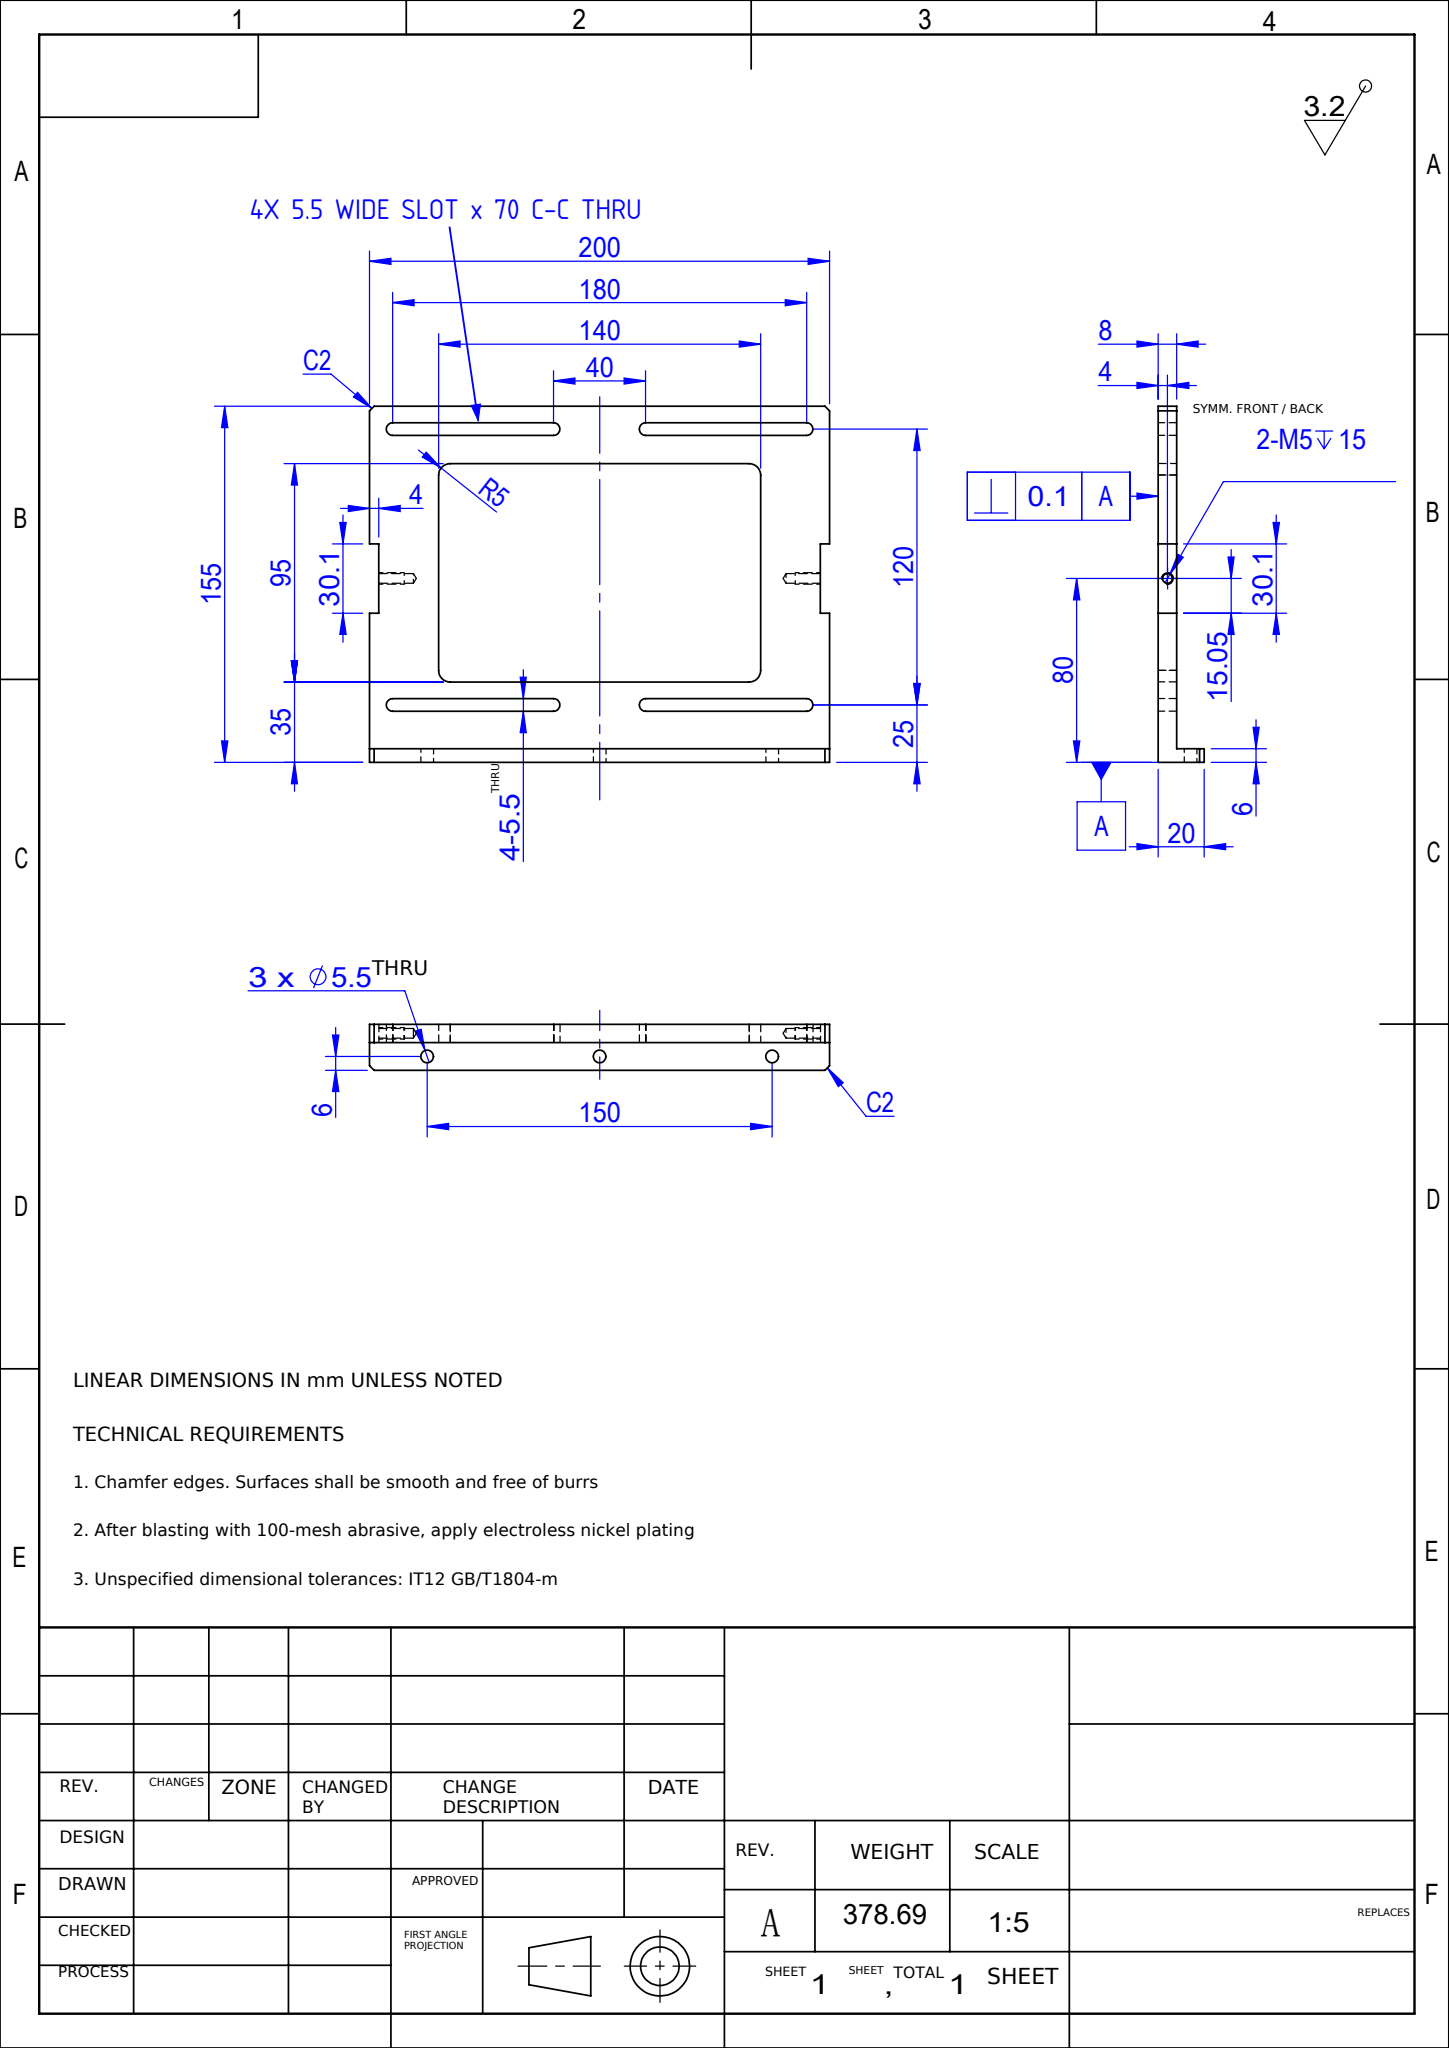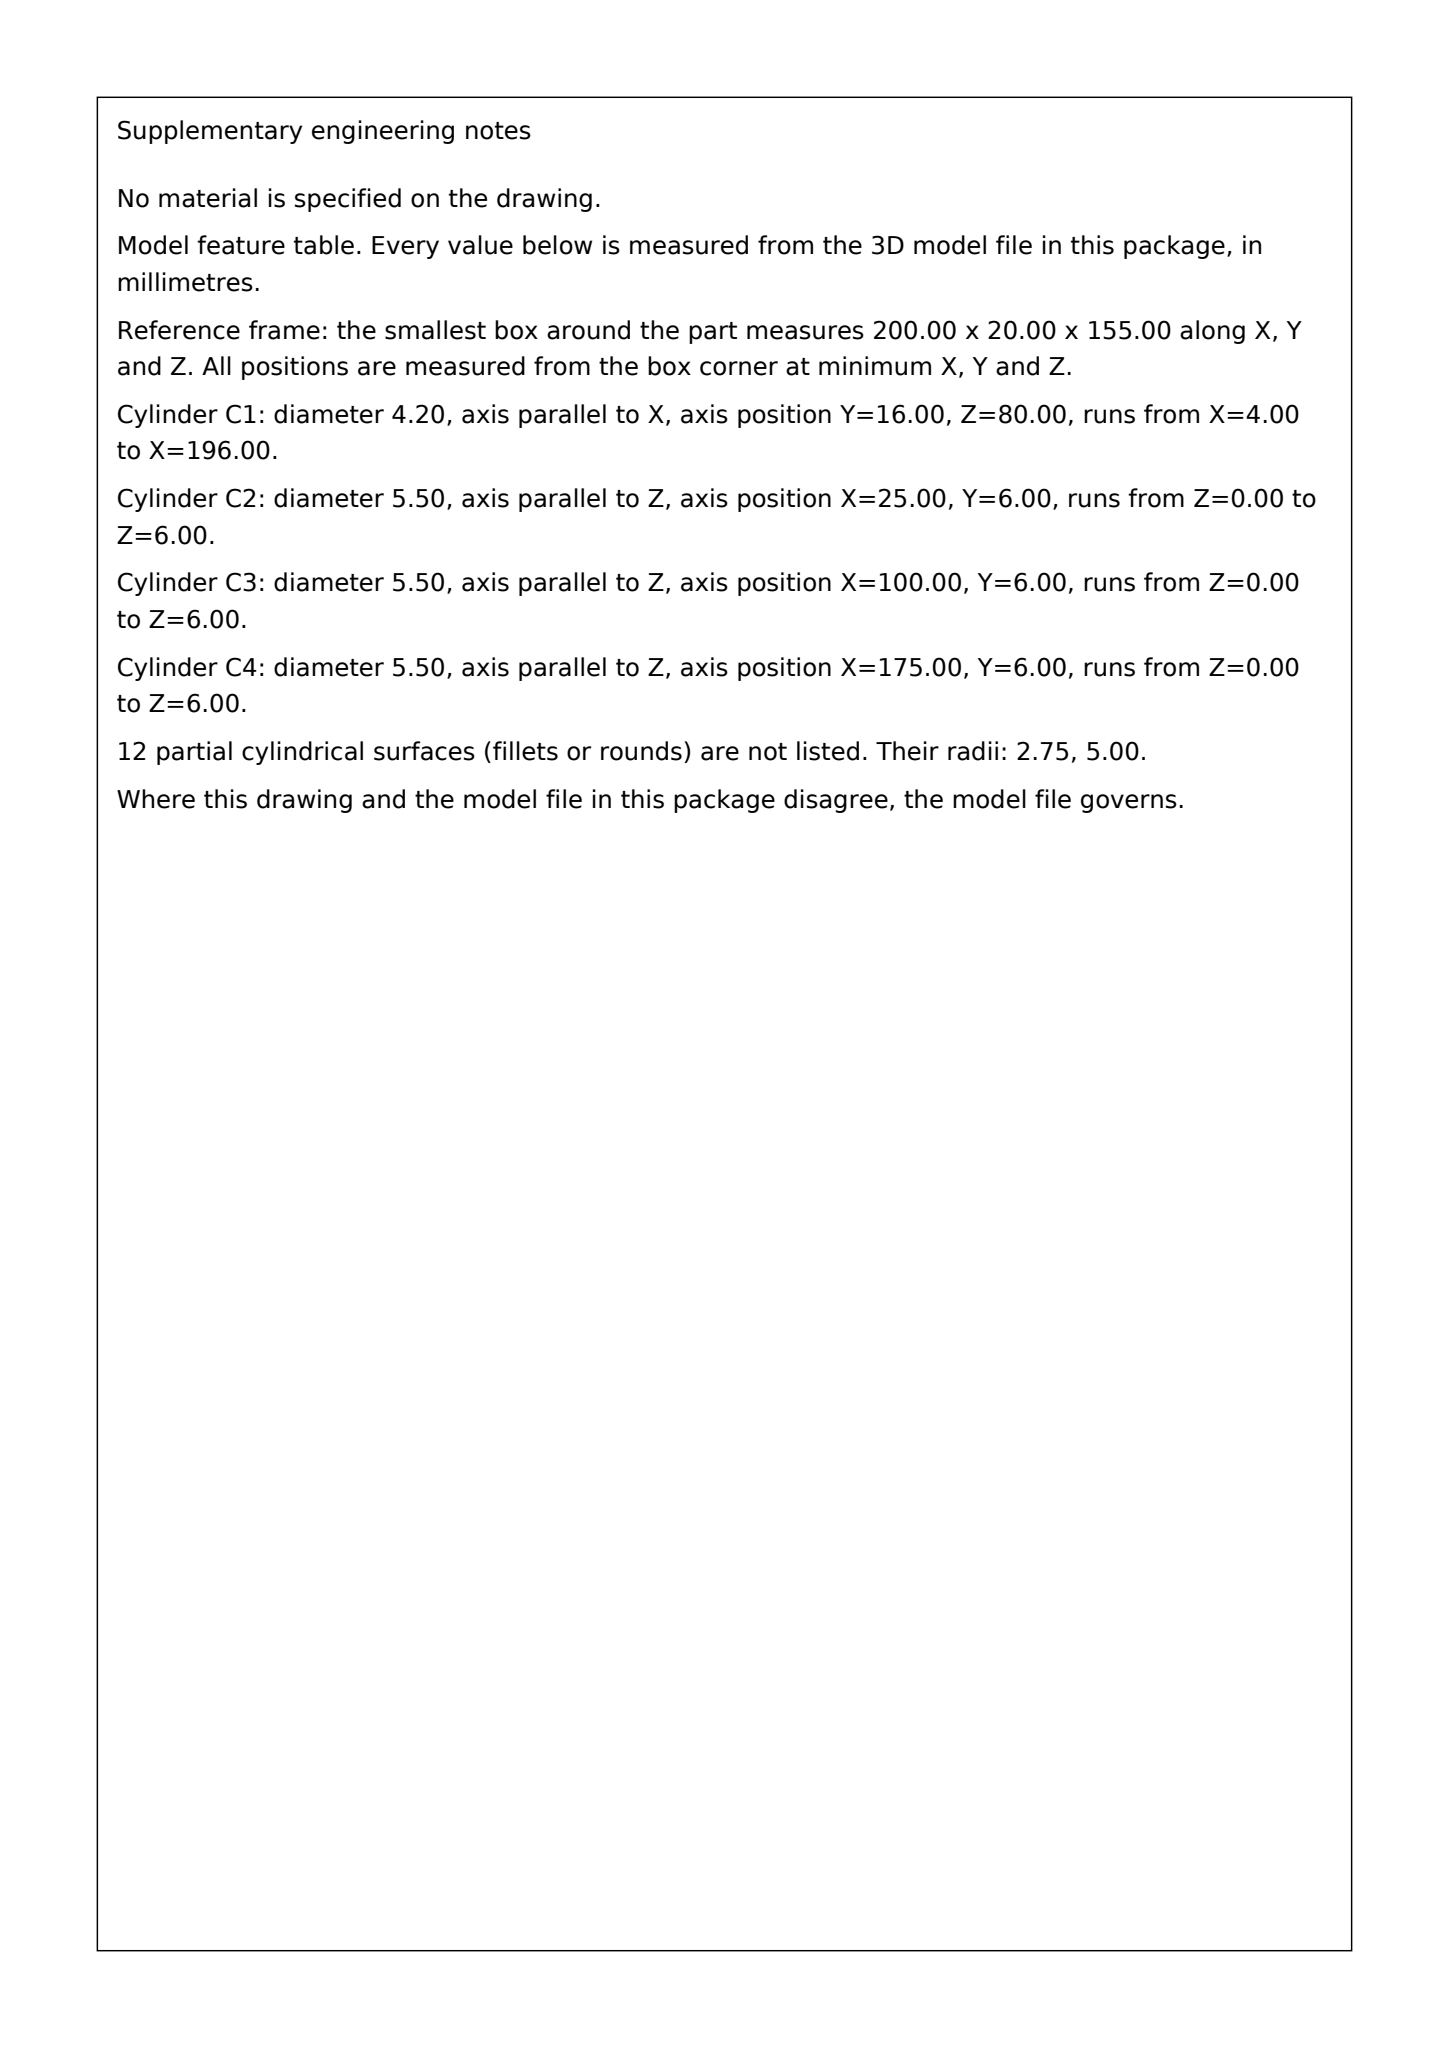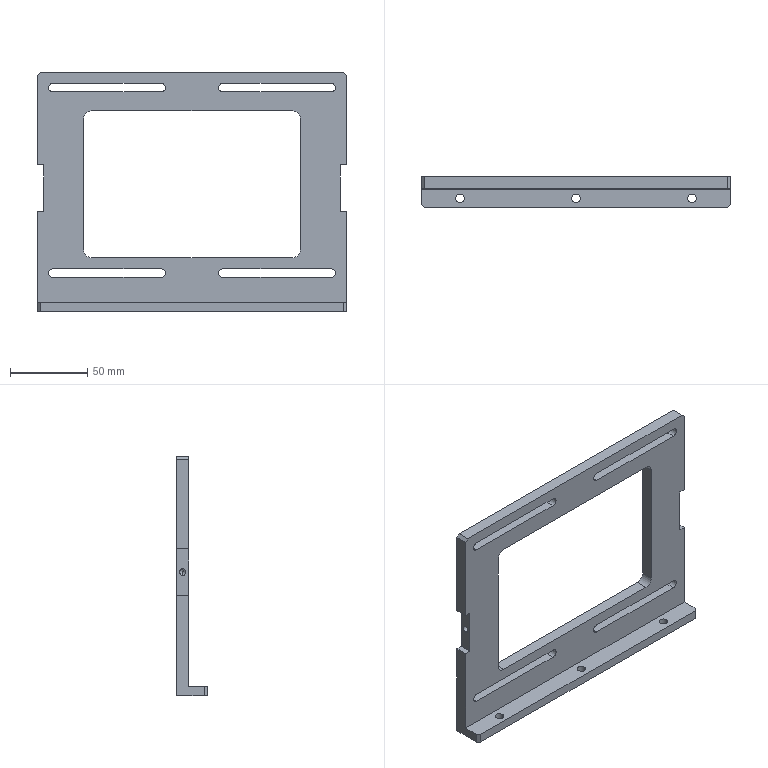Part | SolidWorks | mm | 1 solid | 58 faces | box 200 x 20 x 155 mm | volume 140254 mm3 | plane 32 | cylinder 22 | cone 4 | commonest cylinder face diameters 5.5 x14 4.2 x4 10 x4
Drawing notes:
FRONT VIEW: 4X SLOT 5.5 WIDE x 70 C-C THRU (NOT 4X Ø5.5) | from the solid: Eight 180° arcs Ø5.5 on y-axis at x=10/80 & 120/190, z=145 & 25, from y=12 to 20; planes z=142.2/147.8 and 22.2/27.7 span x 10-80 and 120-190 => 4 slots 5.5 wide, 70 between end centers, thru 8 wall. Separate 3X Ø5.5 thru holes at z-axis x=25,100,175 in 6 base.
build123d program:
from build123d import *

# Parameters (mm, degrees)
SKETCH1_W               = 200
SKETCH1_H               = 8
EXTRUDE1_DEPTH          = 210
FILLET1_R               = 5
SKETCH4_W               = 140
SKETCH4_H               = 155
CUT_EXTRUDE1_DEPTH      = 233.732
SKETCH10_W              = 140
SKETCH10_H              = 25
BOSS_EXTRUDE1_DEPTH     = 8
FILLET2_R               = 5
CUT_EXTRUDE2_DEPTH      = 291.028
CUT_EXTRUDE2_DEPTH_BACK = 291.028
SKETCH16_W              = 400
SKETCH16_H              = 888
CUT_EXTRUDE3_DEPTH      = 233.732
SKETCH17_W              = 200
SKETCH17_H              = 6
BOSS_EXTRUDE2_DEPTH     = 12
M5_CLEARANCE_HOLE2_D    = 5.5
CHAMFER2_SIZE           = 2
SKETCH24_W              = 4
SKETCH24_H              = 30.1
CUT_EXTRUDE4_DEPTH      = 186.54
CUT_EXTRUDE5_DEPTH      = 185.849
LPATTERN2_COUNT         = 2
LPATTERN2_PITCH         = 120
MIRROR3_COPY_1_DEPTH    = 185.849


with BuildPart() as part:
    # Sketch1 → Extrude1 (new body)
    with BuildSketch(Plane.XY):
        Rectangle(SKETCH1_W, SKETCH1_H)
    extrude(amount=EXTRUDE1_DEPTH)

    # Fillet1
    fillet1_edges = [part.edges().sort_by_distance(p)[0] for p in [
        (100, 0, 210),
        (-100, 0, 210),
    ]]
    fillet(fillet1_edges, radius=FILLET1_R)

    # Sketch4 → Cut-Extrude1 (cut, through all)
    with BuildSketch(Plane(origin=(0, 4, 0), x_dir=(1, 0, 0), z_dir=(0, 1, 0))):
        with Locations((0, -112.5)):
            Rectangle(SKETCH4_W, SKETCH4_H)
    extrude(amount=-CUT_EXTRUDE1_DEPTH, mode=Mode.SUBTRACT)

    # Sketch10 → Boss-Extrude1 (add)
    with BuildSketch(Plane.XZ.offset(4)):
        with Locations((0, 142.5)):
            Rectangle(SKETCH10_W, SKETCH10_H)
    extrude(amount=-BOSS_EXTRUDE1_DEPTH)

    # Fillet2
    fillet2_edges = [part.edges().sort_by_distance(p)[0] for p in [
        (-70, 0, 35),
        (70, 0, 35),
        (-70, 0, 130),
        (-70, 0, 155),
        (70, 0, 155),
        (70, 0, 130),
    ]]
    fillet(fillet2_edges, radius=FILLET2_R)

    # Sketch11 → Cut-Extrude2 (cut, two sides: drawn at the far end of the back side and taken through both)
    with BuildSketch(Plane.ZY.offset(100).offset(-CUT_EXTRUDE2_DEPTH_BACK)):
        Polygon((-232.506, 79.381), (195, 4), (211.991, 1.004), (639.498, -74.377), (790.259, 780.635), (-81.744, 934.393), align=None)
    extrude(amount=CUT_EXTRUDE2_DEPTH + CUT_EXTRUDE2_DEPTH_BACK, mode=Mode.SUBTRACT)

    # Sketch16 → Cut-Extrude3 (cut, through all)
    with BuildSketch(Plane(origin=(0, 4, 0), x_dir=(1, 0, 0), z_dir=(0, 1, 0))):
        with Locations((100, -599)):
            Rectangle(SKETCH16_W, SKETCH16_H)
    extrude(amount=-CUT_EXTRUDE3_DEPTH, mode=Mode.SUBTRACT)

    # Sketch17 → Boss-Extrude2 (add)
    with BuildSketch(Plane.XZ.offset(4)):
        with Locations((0, 3)):
            Rectangle(SKETCH17_W, SKETCH17_H)
    extrude(amount=BOSS_EXTRUDE2_DEPTH)

    # M5 Clearance Hole2 (through all)
    with Locations(Plane(origin=(124.661, 0.05817, 6), x_dir=(-1, 0, 0), z_dir=(0, 0, 1))):
        with Locations((49.661, 10.058), (124.661, 10.058), (199.661, 10.058)):
            Hole(M5_CLEARANCE_HOLE2_D / 2)

    # Chamfer2
    chamfer2_edges = [part.edges().sort_by_distance(p)[0] for p in [
        (-100, -16, 3),
        (100, -16, 3),
        (100, 0, 155),
        (-100, 0, 155),
    ]]
    chamfer(chamfer2_edges, length=CHAMFER2_SIZE)

    # Sketch22 → M5 Tapped Hole3 (revolve, cut)
    with BuildSketch(Plane(origin=(100, 0, 80), x_dir=(0, 0, -1), z_dir=(0, 1, 0))):
        Polygon((0, 0), (0, 20.262), (2.1, 19), (2.1, 0), align=None)
    m5_tapped_hole3 = revolve(axis=Axis((106.35, 0, 80), (-1, 0, 0)), mode=Mode.SUBTRACT)

    # Mirror2: M5 Tapped Hole3 across plane
    add(m5_tapped_hole3.mirror(Plane(origin=(0, 0, 0), x_dir=(0, 0, 1), z_dir=(1, 0, 0))), mode=Mode.SUBTRACT)

    # Sketch24 → Cut-Extrude4 (cut, through all)
    with BuildSketch(Plane(origin=(0, 4, 0), x_dir=(1, 0, 0), z_dir=(0, 1, 0))):
        with Locations((-98, -80)):
            Rectangle(SKETCH24_W, SKETCH24_H)
        with Locations((98, -80)):
            Rectangle(SKETCH24_W, SKETCH24_H)
    extrude(amount=-CUT_EXTRUDE4_DEPTH, mode=Mode.SUBTRACT)

    # Sketch25 → Cut-Extrude5 (cut, through all)
    with BuildSketch(Plane.XZ.offset(4)):
        with BuildLine():
            Line((-90, 147.75), (-20, 147.75))
            ThreePointArc((-20, 147.75), (-17.25, 145), (-20, 142.25))
            Line((-20, 142.25), (-90, 142.25))
            ThreePointArc((-90, 142.25), (-92.75, 145), (-90, 147.75))
        make_face()
    cut_extrude5 = extrude(amount=-CUT_EXTRUDE5_DEPTH, mode=Mode.SUBTRACT)

    # LPattern2: Cut-Extrude5 ×2
    with Locations(*[(0, 0, -i * LPATTERN2_PITCH) for i in range(1, LPATTERN2_COUNT)]):
        add(cut_extrude5, mode=Mode.SUBTRACT)

    # Mirror3: Cut-Extrude5 across plane
    add(cut_extrude5.mirror(Plane(origin=(0, 0, 0), x_dir=(0, 0, 1), z_dir=(1, 0, 0))), mode=Mode.SUBTRACT)

    # Mirror3 copy 1 sketch → Mirror3 copy 1 (cut, through all)
    with BuildSketch(Plane(origin=(0, -4, -120), x_dir=(-1, 0, 0), z_dir=(0, -1, 0))):
        with BuildLine():
            Line((-90, -147.75), (-20, -147.75))
            ThreePointArc((-20, -147.75), (-17.25, -145), (-20, -142.25))
            Line((-20, -142.25), (-90, -142.25))
            ThreePointArc((-90, -142.25), (-92.75, -145), (-90, -147.75))
        make_face()
    extrude(amount=-MIRROR3_COPY_1_DEPTH, mode=Mode.SUBTRACT)


solid = part.part